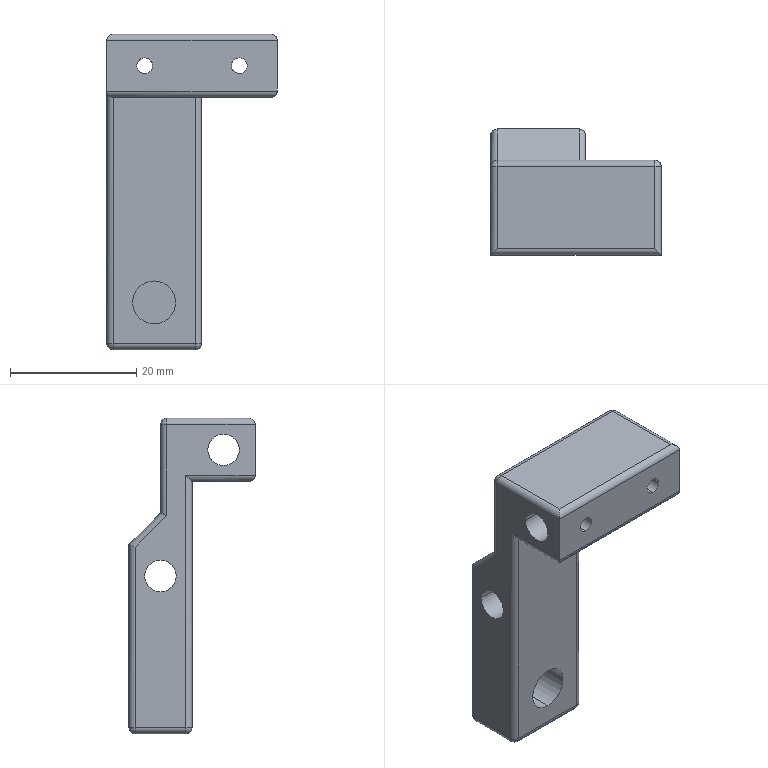Component | SolidWorks | 18ZTJ-NVT-01-004-1 | 1 solid | 57 faces | box 27 x 20 x 50 mm | volume 8260 mm3 | cylinder 37 | plane 13 | sphere 7 | commonest cylinder face diameters 2 x21 2.5 x8 5 x4 4.5 x2 6.8 x2 | material #45